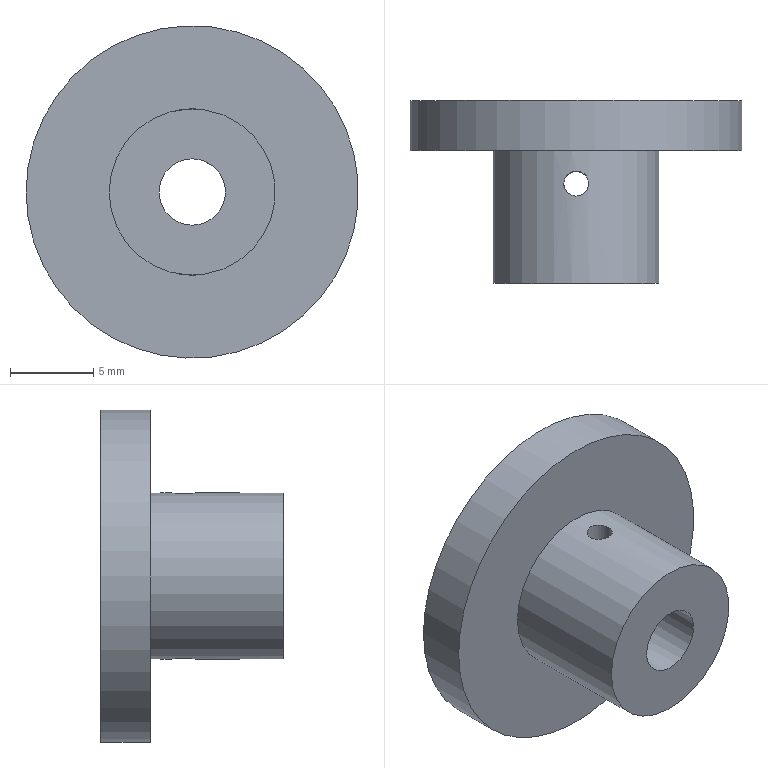Component | NX | HANDLE_1 | 1 solid | 8 faces | volume 1422 mm3 | cylinder 5 | plane 3 | commonest cylinder face diameters 1.5 x2 10 x1 20 x1 4 x1